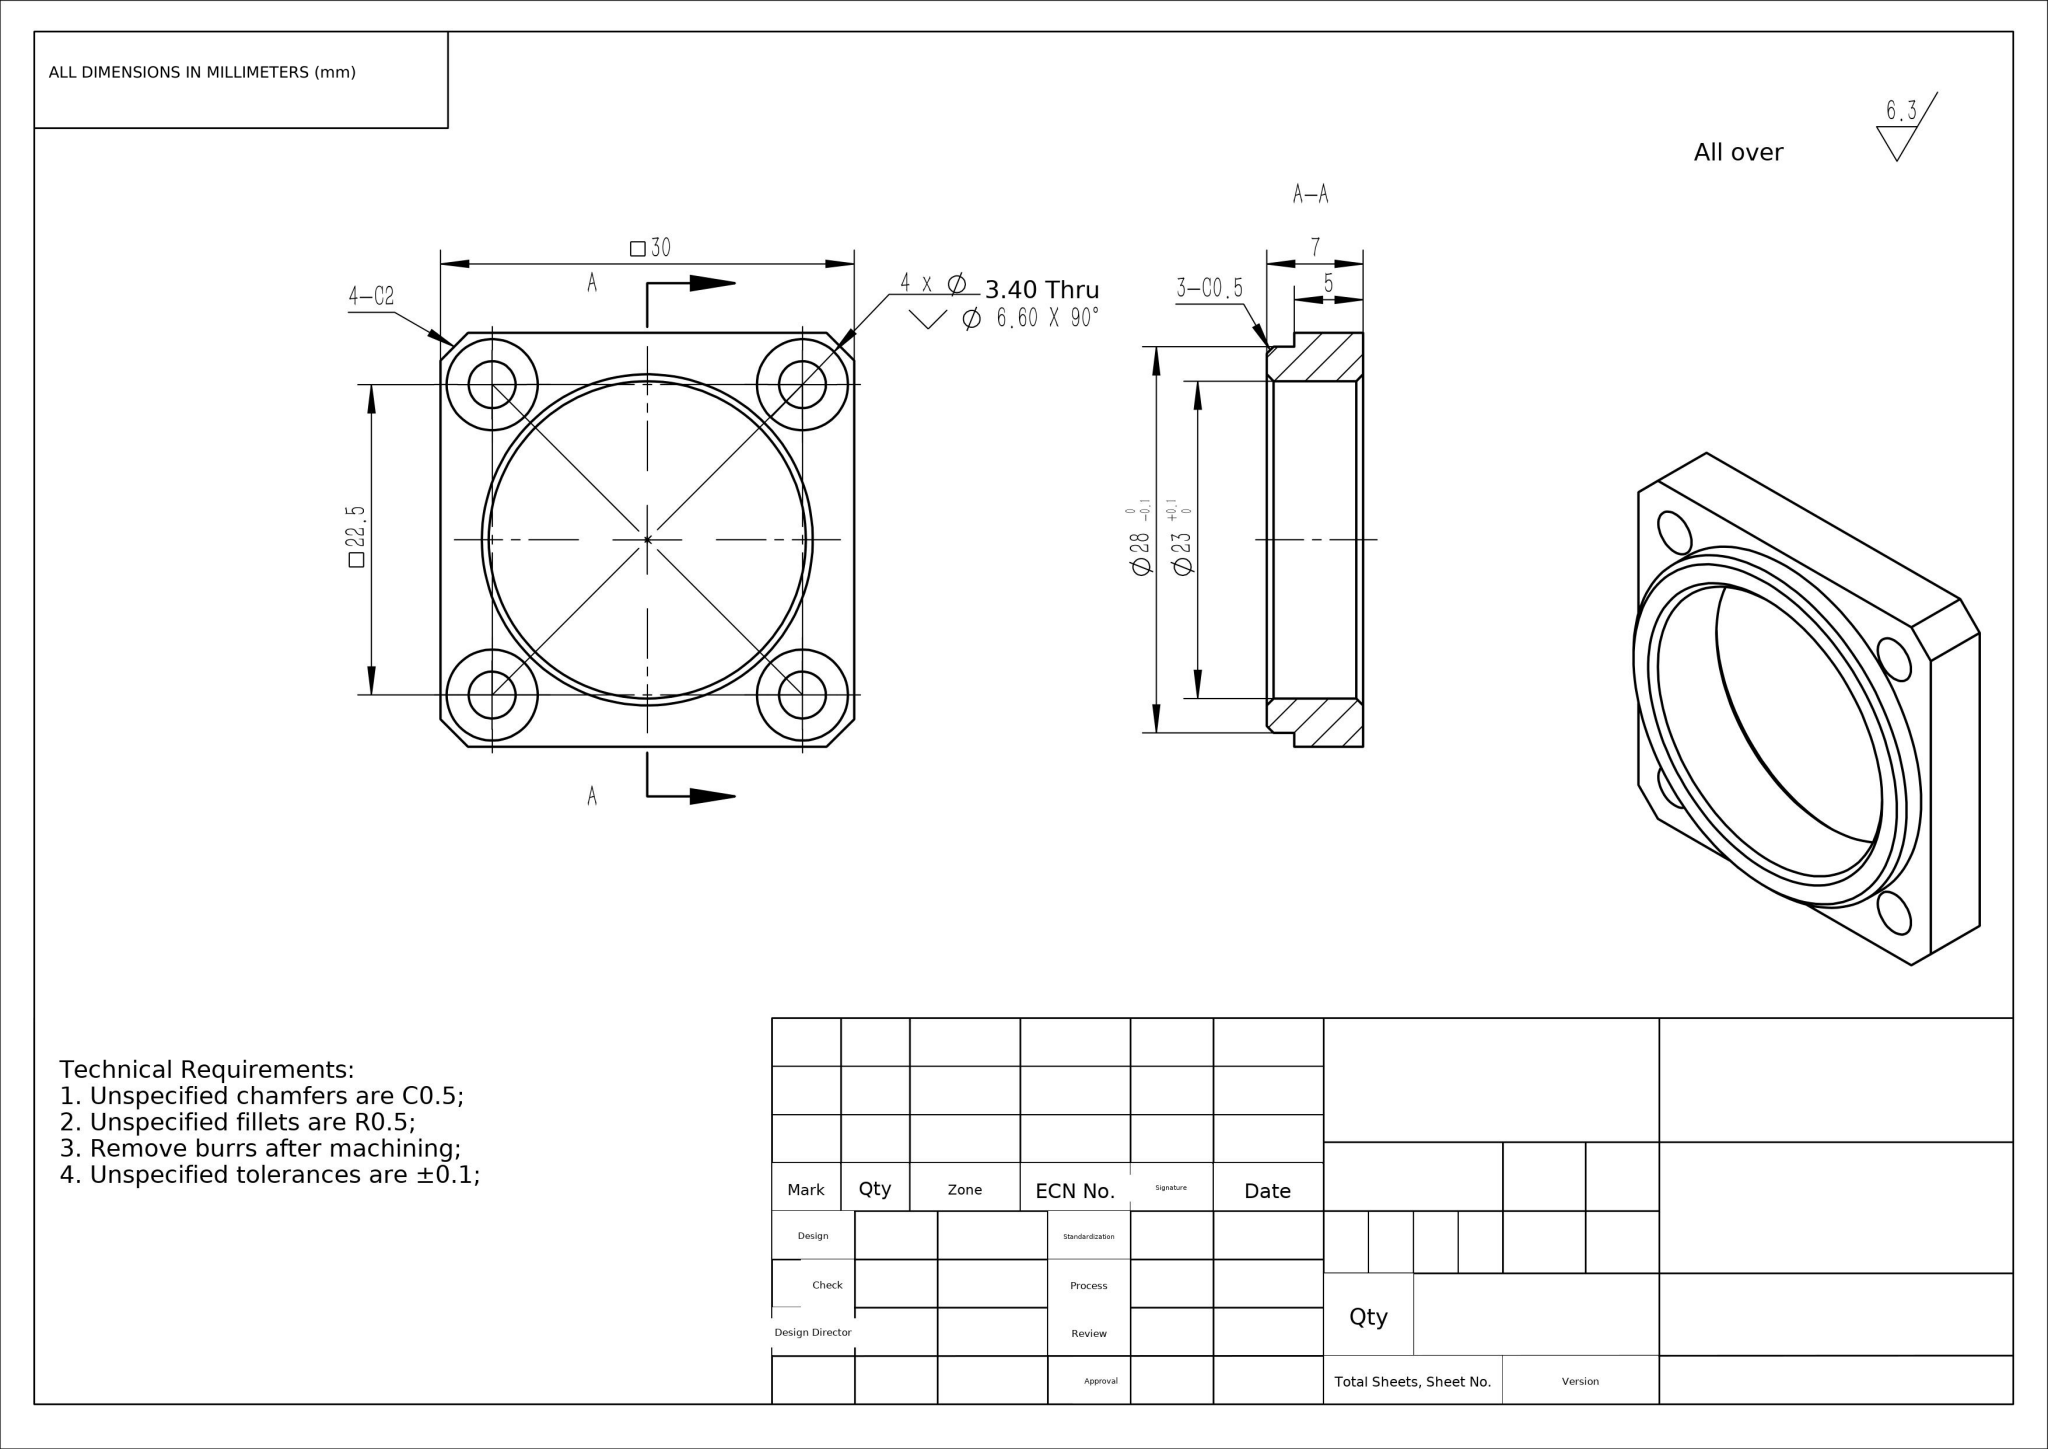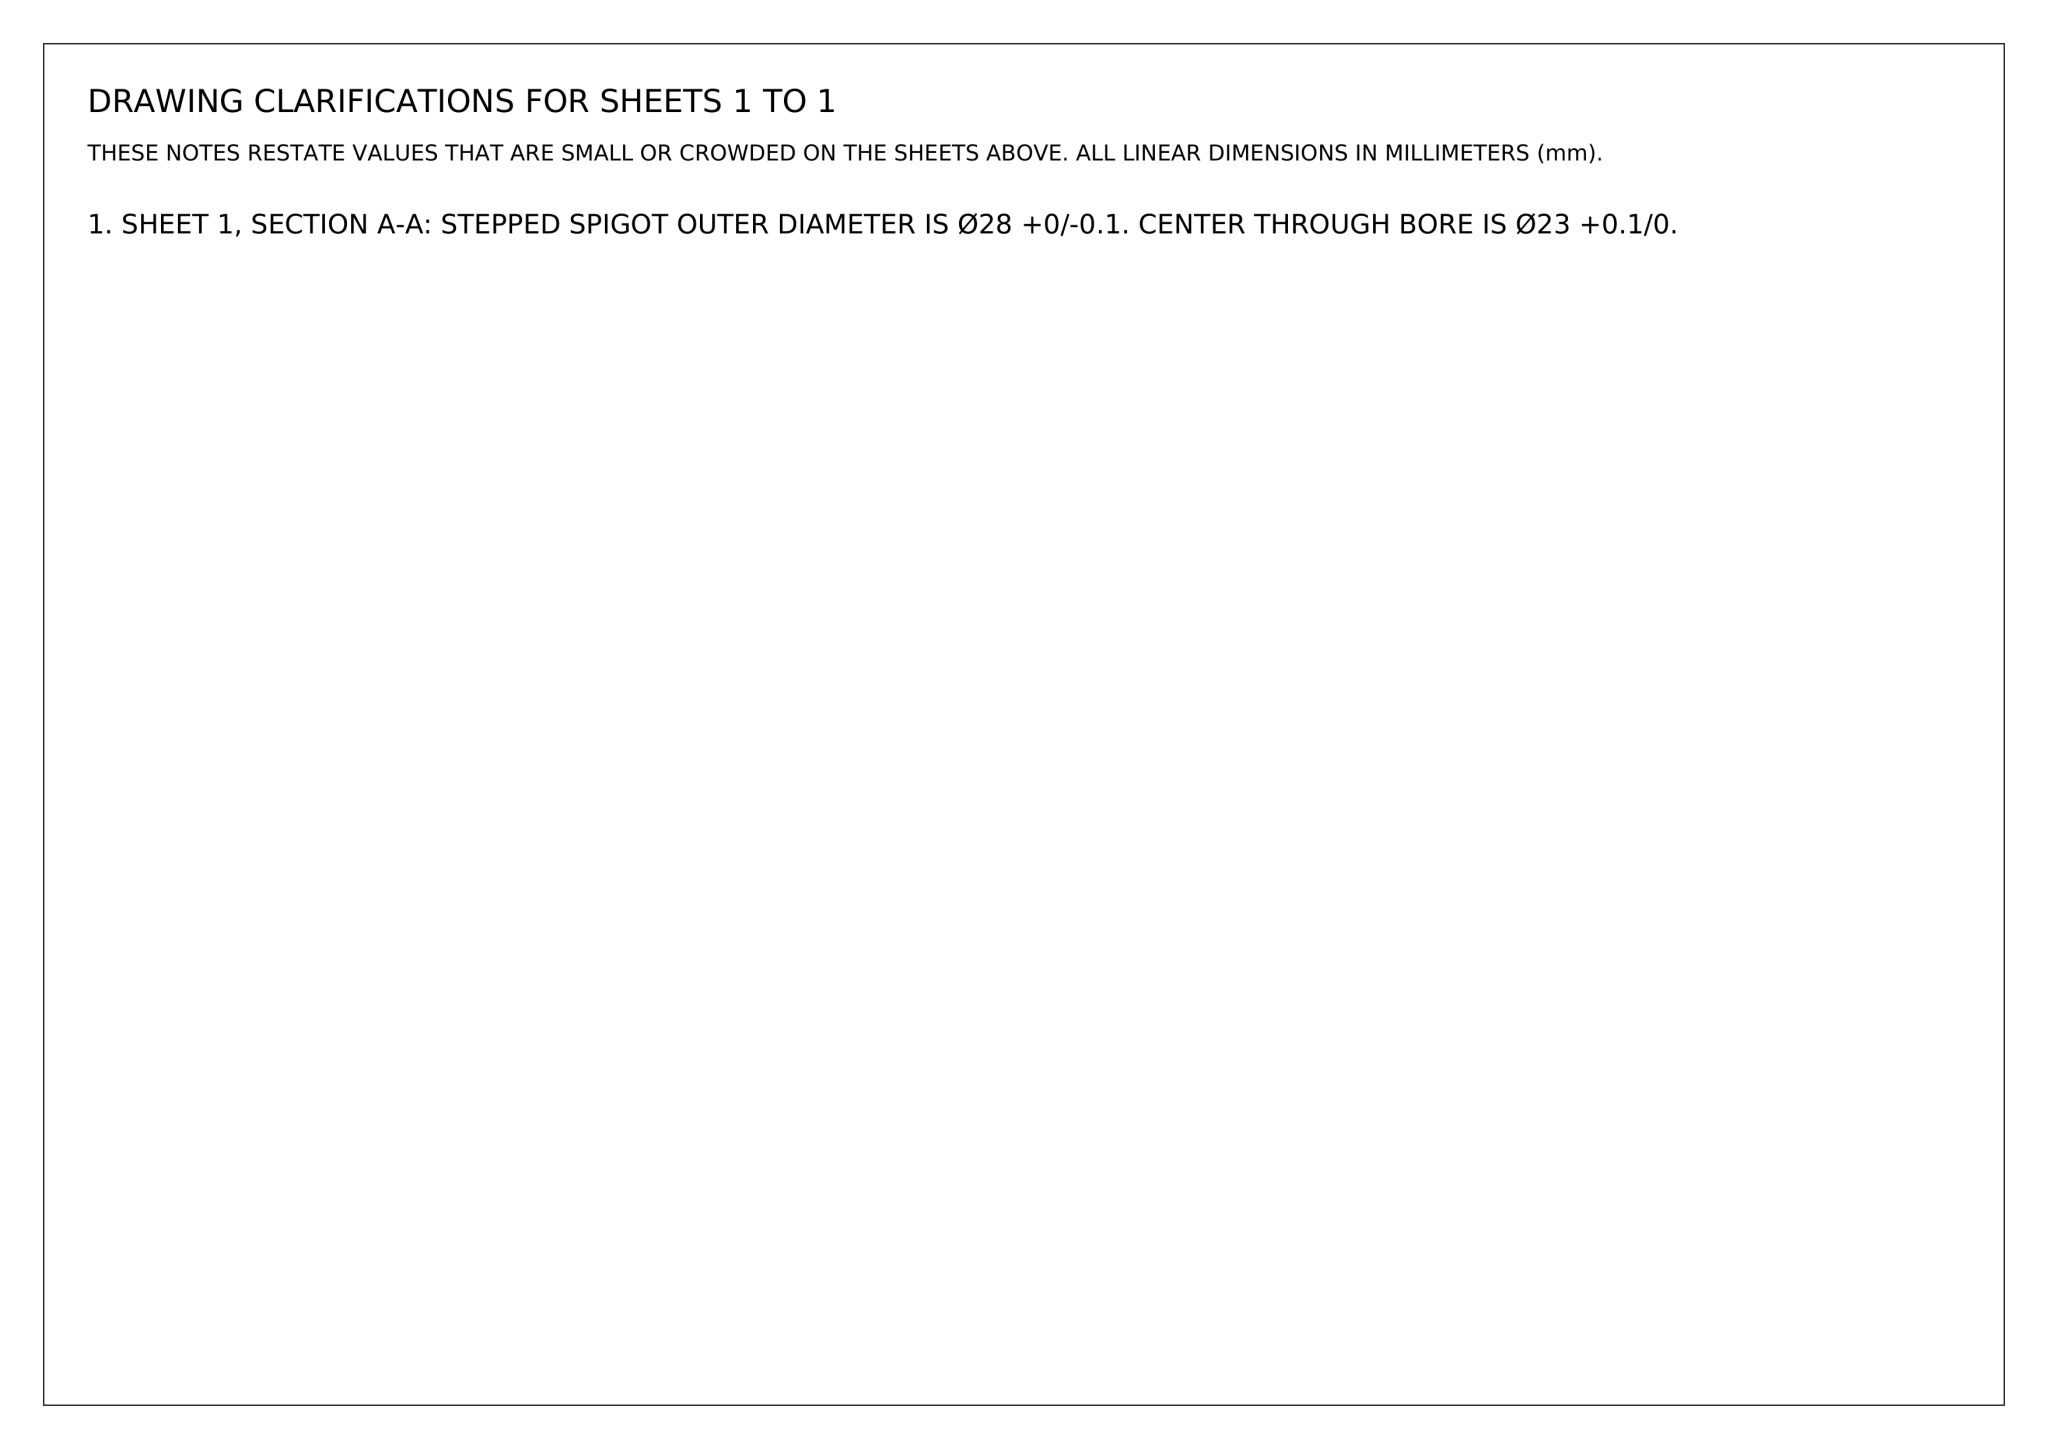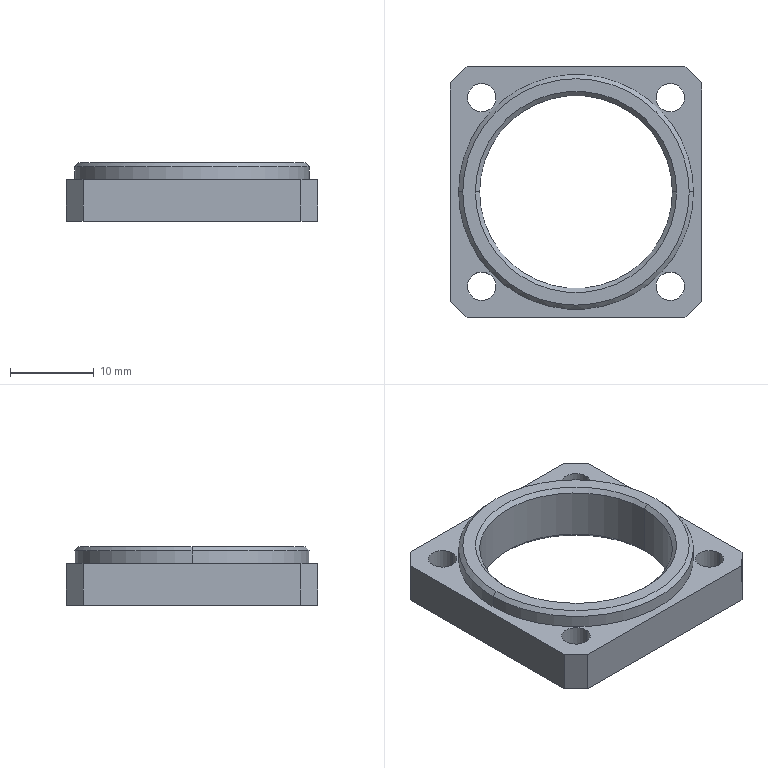Part | NX | mm | 1 solid | 37 faces | box 30 x 30 x 7 mm | volume 2501 mm3 | cone 14 | cylinder 12 | plane 11 | commonest cylinder face diameters 3.4 x8 28 x2 23 x2